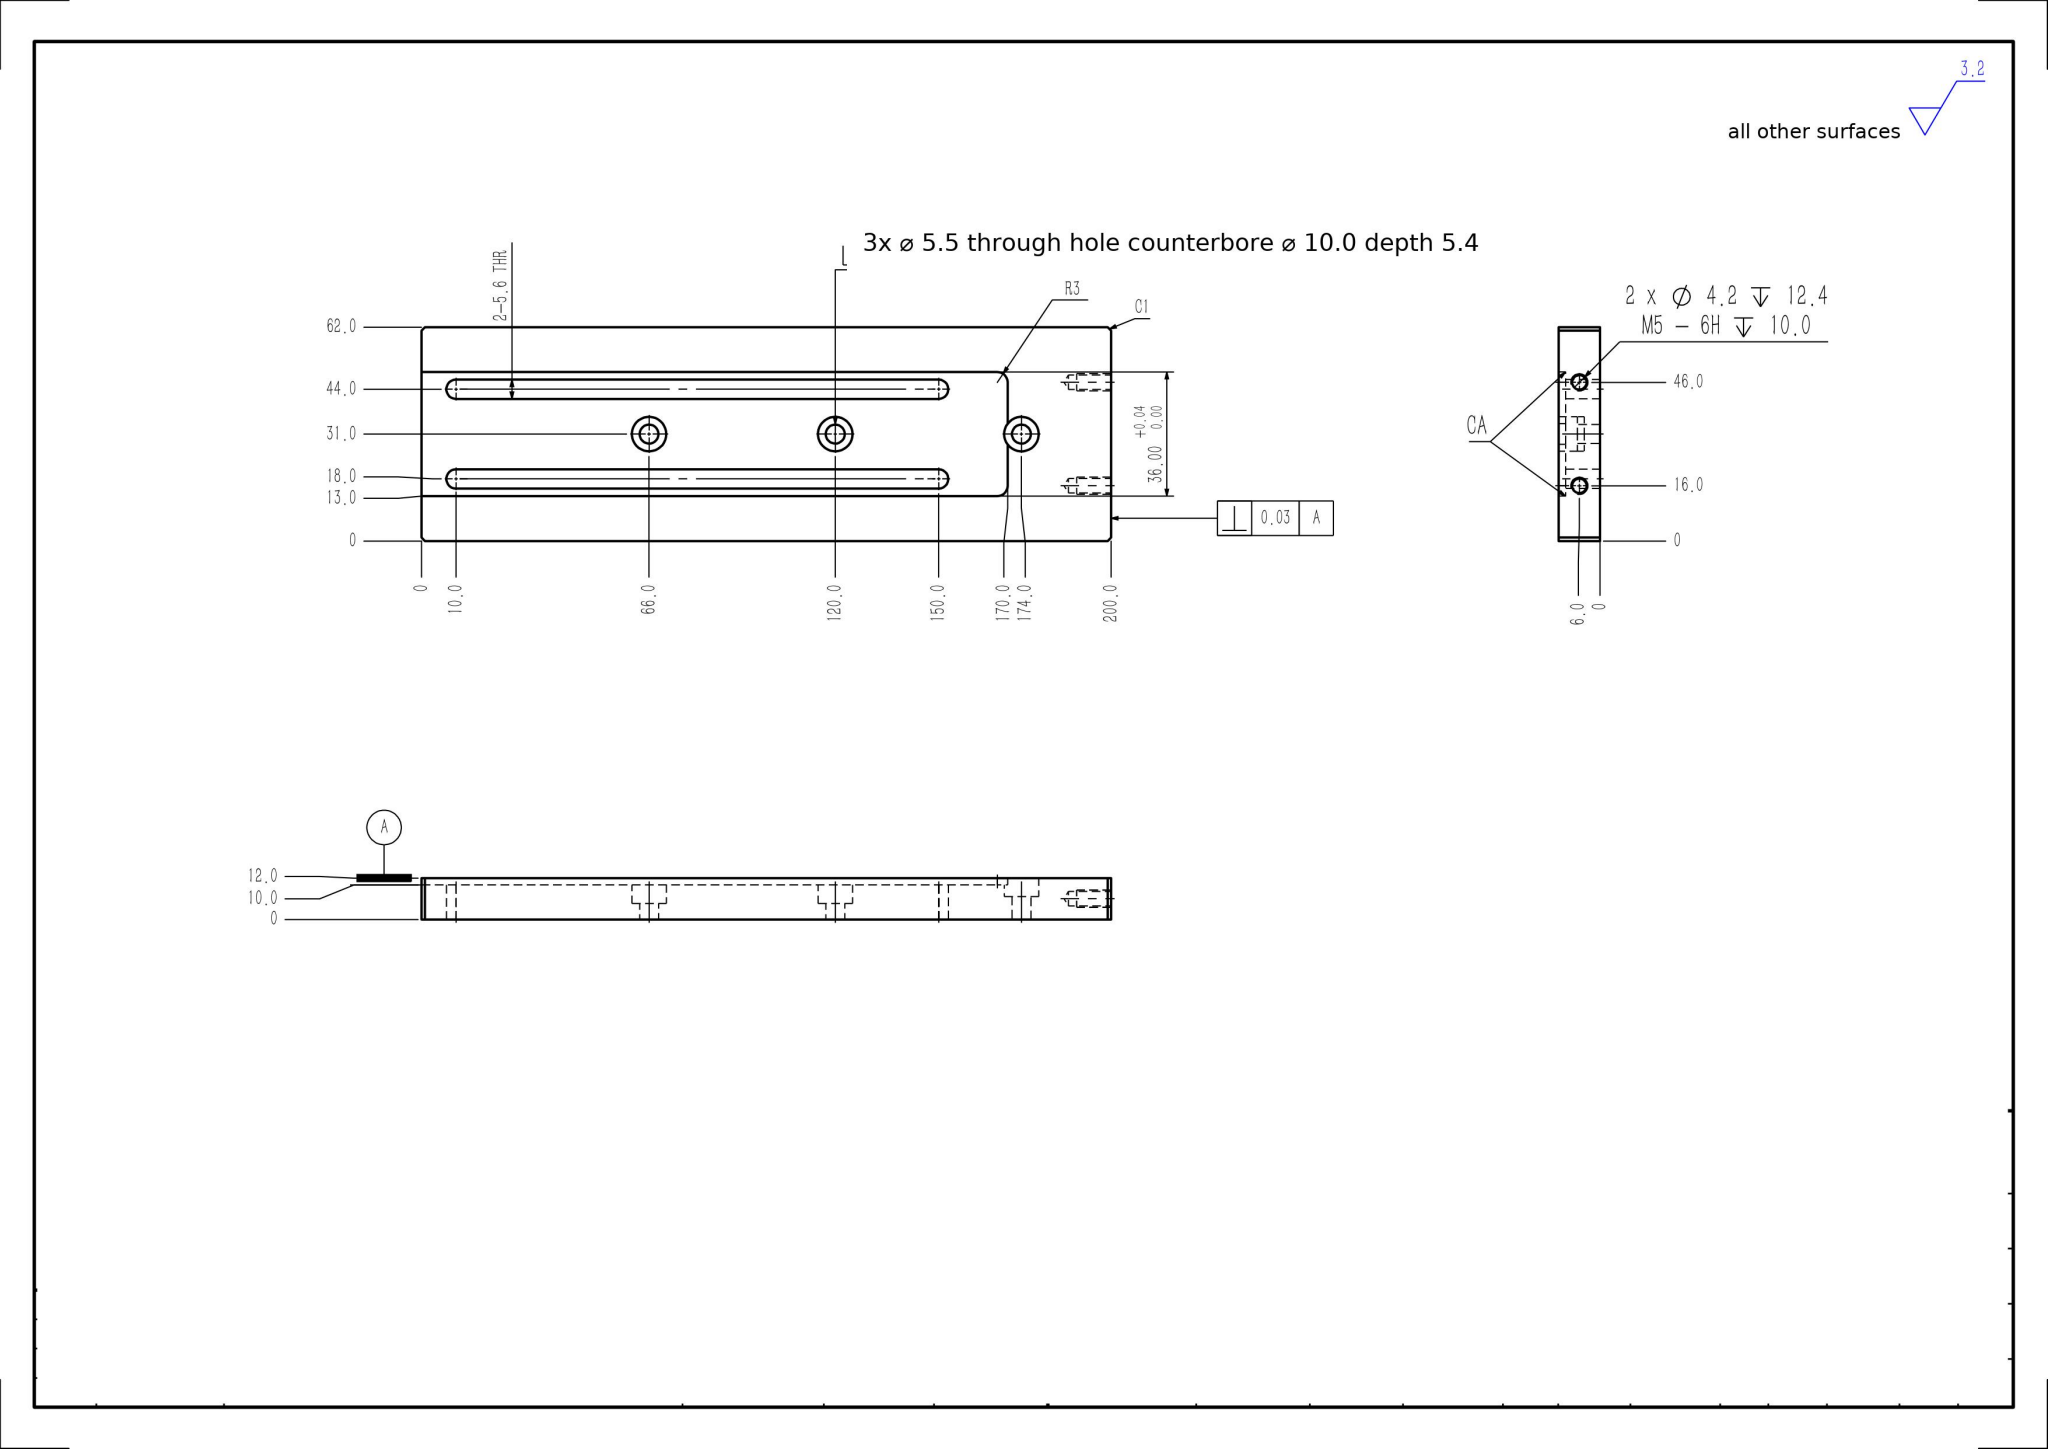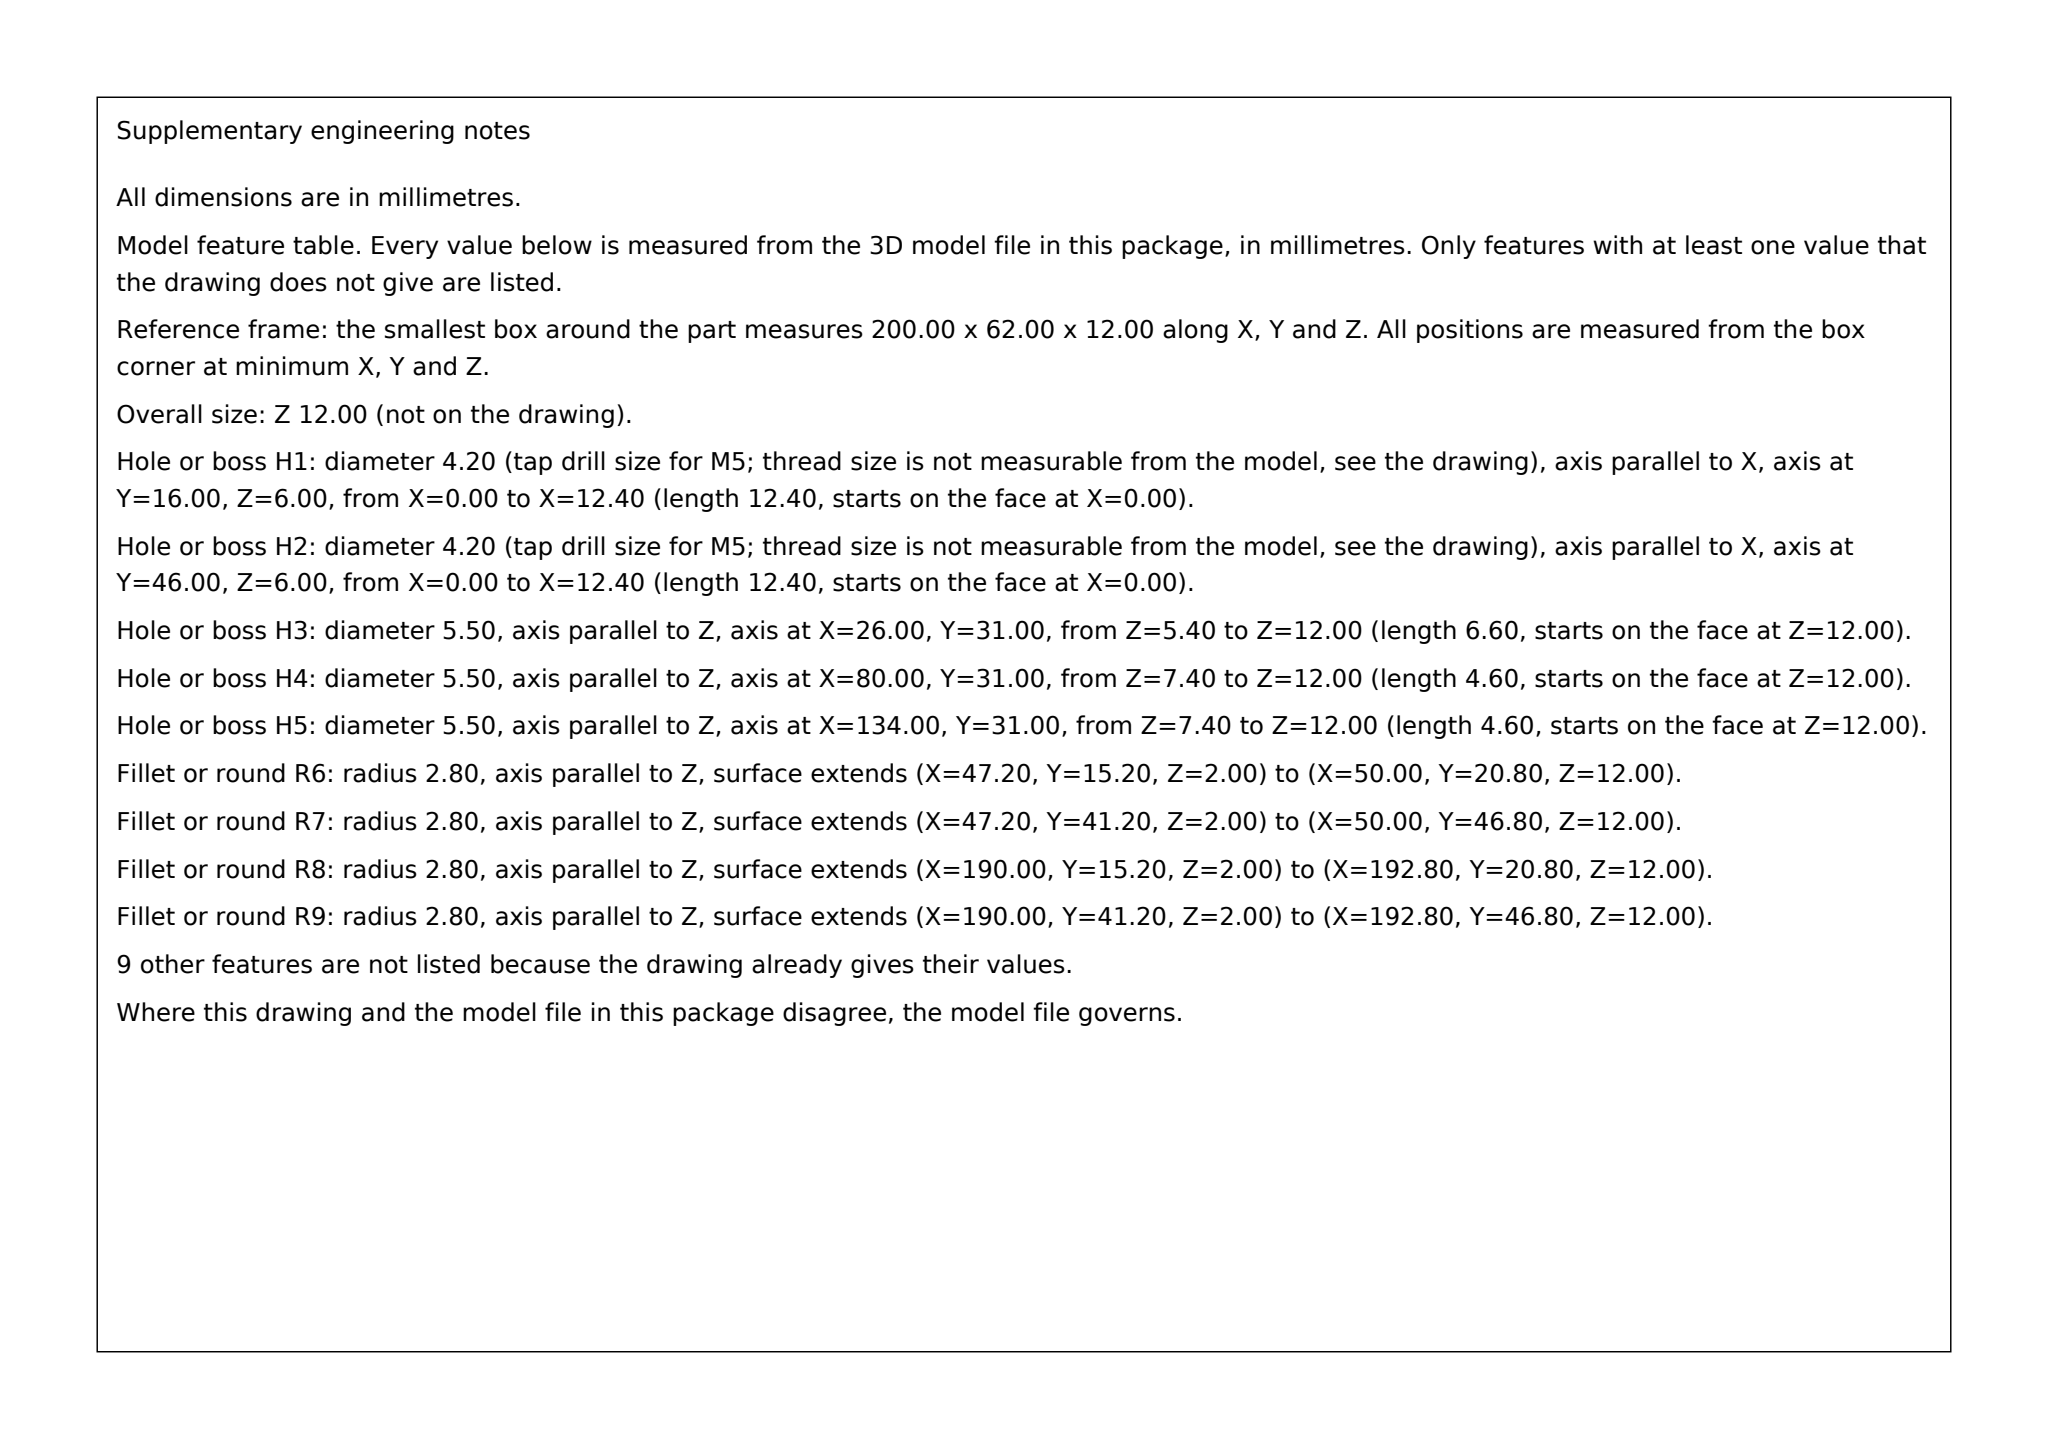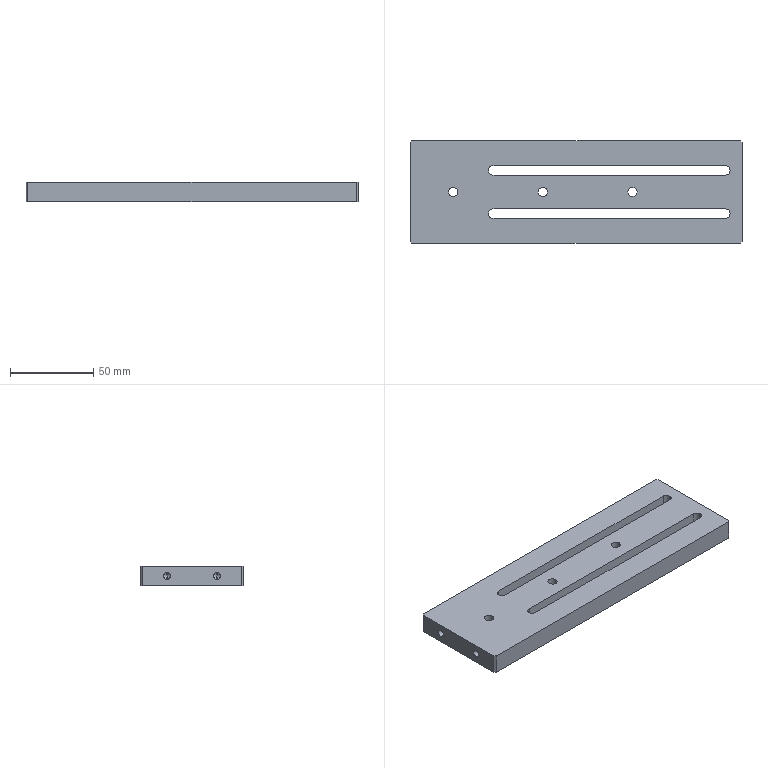Part | SolidWorks | mm | 1 solid | 50 faces | box 200 x 62 x 12 mm | volume 118376 mm3 | cylinder 24 | plane 22 | cone 4 | commonest cylinder face diameters 5.6 x6 5.5 x6 10 x6 4.2 x4 6 x2
build123d program:
from build123d import *

# Parameters (mm, degrees)
SKETCH1_W                                       = 200
SKETCH1_H                                       = 62
BOSS_EXTRUDE1_DEPTH                             = 6
CUT_EXTRUDE1_DEPTH                              = 2
M5_TAPPED_HOLE1_D                               = 4.2
M5_TAPPED_HOLE1_DEPTH                           = 12.4
M5_TAPPED_HOLE1_TIP                             = 1.262
M5_HEX_SOCKET_HEAD_CAP_SCREW_CBORE1_D           = 5.5
M5_HEX_SOCKET_HEAD_CAP_SCREW_CBORE1_CBORE_D     = 10
M5_HEX_SOCKET_HEAD_CAP_SCREW_CBORE1_CBORE_DEPTH = 5.4
M5_HEX_SOCKET_HEAD_CAP_SCREW_CBORE2_D           = 5.5
M5_HEX_SOCKET_HEAD_CAP_SCREW_CBORE2_CBORE_D     = 10
M5_HEX_SOCKET_HEAD_CAP_SCREW_CBORE2_CBORE_DEPTH = 5.4
CUT_EXTRUDE2_DEPTH                              = 106.38
CHAMFER1_SIZE                                   = 1


with BuildPart() as part:
    # Sketch1 → Boss-Extrude1 (new, symmetric)
    with BuildSketch(Plane.XY):
        Rectangle(SKETCH1_W, SKETCH1_H)
    extrude(amount=BOSS_EXTRUDE1_DEPTH, both=True)

    # Sketch2 → Cut-Extrude1 (cut)
    with BuildSketch(Plane(origin=(0, 0, -6), x_dir=(-1, 0, 0), z_dir=(0, 0, -1))):
        with BuildLine():
            Line((-100, -18), (67, -18))
            ThreePointArc((67, -18), (69.121, -17.121), (70, -15))
            Line((70, -15), (70, 15))
            ThreePointArc((70, 15), (69.121, 17.121), (67, 18))
            Line((67, 18), (-100, 18))
            Line((-100, 18), (-100, -18))
        make_face()
    extrude(amount=-CUT_EXTRUDE1_DEPTH, mode=Mode.SUBTRACT)

    # M5 Tapped Hole1
    with Locations(Plane.ZY.offset(100)):
        with Locations((0, 15), (0, -15)):
            Hole(M5_TAPPED_HOLE1_D / 2, depth=M5_TAPPED_HOLE1_DEPTH)
            with Locations((0, 0, -(M5_TAPPED_HOLE1_DEPTH + M5_TAPPED_HOLE1_TIP / 2))):  # 118° drill point
                Cone(0, M5_TAPPED_HOLE1_D / 2, M5_TAPPED_HOLE1_TIP, mode=Mode.SUBTRACT)

    # M5 Hex Socket Head Cap Screw CBORE1 (through all)
    with Locations(Plane(origin=(0, 0, -4), x_dir=(-1, 0, 0), z_dir=(0, 0, -1))):
        with Locations((-34, 0), (20, 0)):
            CounterBoreHole(M5_HEX_SOCKET_HEAD_CAP_SCREW_CBORE1_D / 2, M5_HEX_SOCKET_HEAD_CAP_SCREW_CBORE1_CBORE_D / 2, M5_HEX_SOCKET_HEAD_CAP_SCREW_CBORE1_CBORE_DEPTH)

    # M5 Hex Socket Head Cap Screw CBORE2 (through all)
    with Locations(Plane(origin=(0, 0, -6), x_dir=(-1, 0, 0), z_dir=(0, 0, -1))):
        with Locations((74, 0)):
            CounterBoreHole(M5_HEX_SOCKET_HEAD_CAP_SCREW_CBORE2_D / 2, M5_HEX_SOCKET_HEAD_CAP_SCREW_CBORE2_CBORE_D / 2, M5_HEX_SOCKET_HEAD_CAP_SCREW_CBORE2_CBORE_DEPTH)

    # Sketch9 → Cut-Extrude2 (cut, through all)
    with BuildSketch(Plane.XY.offset(6)):
        with BuildLine():
            Line((90, -15.8), (-50, -15.8))
            ThreePointArc((-50, -15.8), (-52.8, -13), (-50, -10.2))
            Line((-50, -10.2), (90, -10.2))
            ThreePointArc((90, -10.2), (92.8, -13), (90, -15.8))
        make_face()
        with BuildLine():
            Line((90, 15.8), (-50, 15.8))
            ThreePointArc((-50, 15.8), (-52.8, 13), (-50, 10.2))
            Line((-50, 10.2), (90, 10.2))
            ThreePointArc((90, 10.2), (92.8, 13), (90, 15.8))
        make_face()
    extrude(amount=-CUT_EXTRUDE2_DEPTH, mode=Mode.SUBTRACT)

    # Chamfer1
    chamfer1_edges = [part.edges().sort_by_distance(p)[0] for p in [
        (100, -31, 0),
        (-100, -31, 0),
        (-100, 31, 0),
        (100, 31, 0),
    ]]
    chamfer(chamfer1_edges, length=CHAMFER1_SIZE)


solid = part.part